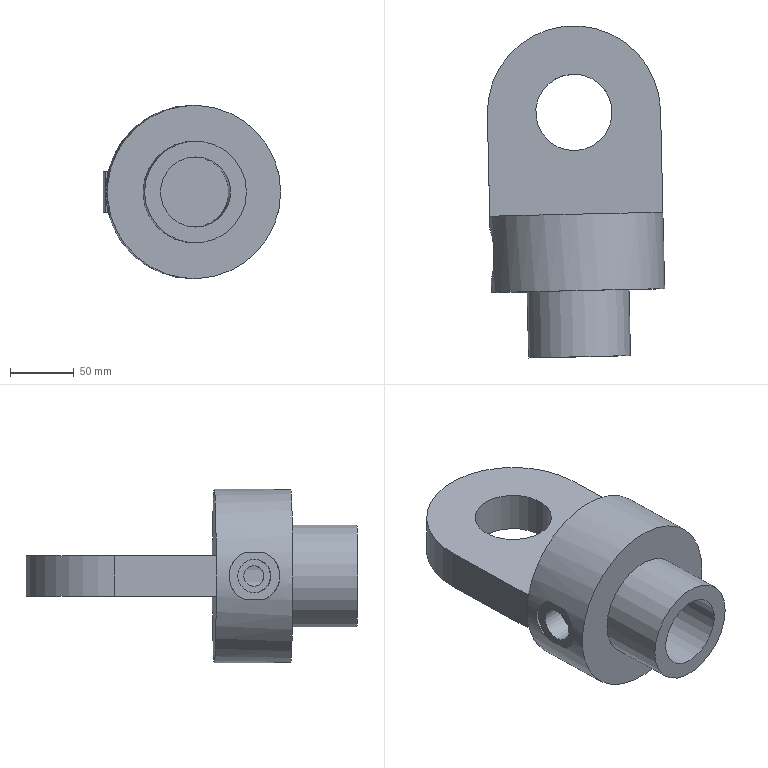Component | NX | 1 | 1 solid | 26 faces | volume 1299897 mm3 | plane 16 | cylinder 10 | commonest cylinder face diameters 136 x2 40 x2 55 x1 80 x1 75 x1 60 x1 26 x1 16 x1